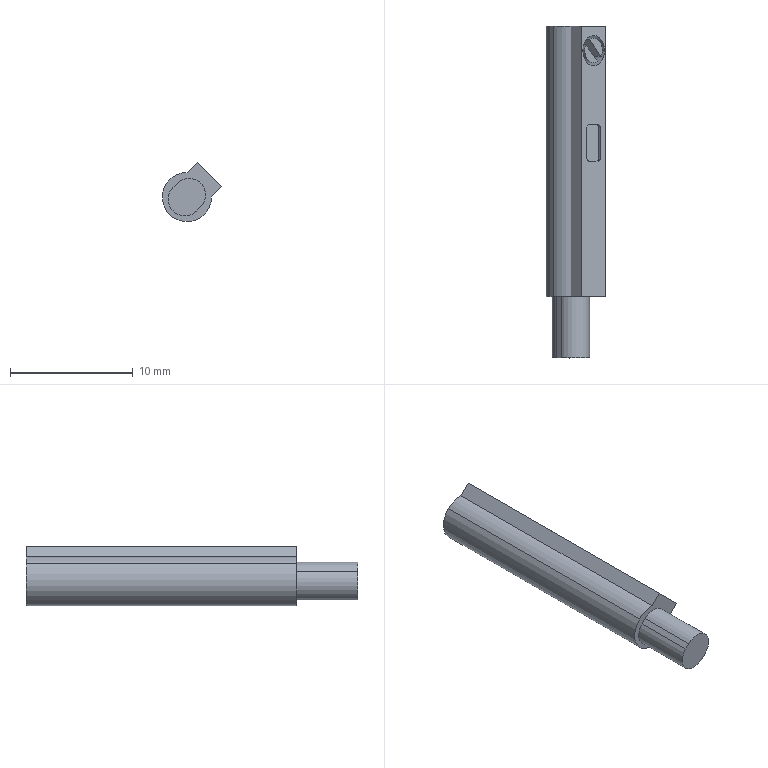Component | SolidWorks | BearingLiftingModule-1_CylinderLiftingModule-1_CDQ2B20-40DZ-L-M9B_0_0_0-1_D-M9B(CQ2_20)-1 | 1 solid | 32 faces | box 4.83 x 27 x 4.83 mm | volume 355 mm3 | plane 19 | cylinder 13 | commonest cylinder face diameters 0.6 x4 4 x3 2 x2 2.5 x2 2.7 x2
STEP:
#1=COLOUR_RGB('',0.7922,0.8196,0.9333);
#2=FILL_AREA_STYLE_COLOUR('',#1);
#3=FILL_AREA_STYLE('',(#2));
#4=SURFACE_STYLE_FILL_AREA(#3);
#5=SURFACE_SIDE_STYLE('',(#4));
#6=SURFACE_STYLE_USAGE(.BOTH.,#5);
#7=PRESENTATION_STYLE_ASSIGNMENT((#6));
#8=CARTESIAN_POINT('',(3.187,-4.024,1.713));
#9=VERTEX_POINT('',#8);
#10=CARTESIAN_POINT('',(3.147,-3.989,1.754));
#11=VERTEX_POINT('',#10);
#12=CARTESIAN_POINT('',(3.16,-4.024,1.741));
#13=DIRECTION('',(0.7071,0.,0.7071));
#14=DIRECTION('',(0.,-1.,0.));
#15=AXIS2_PLACEMENT_3D('',#12,#13,#14);
#16=CIRCLE('',#15,0.03937);
#17=EDGE_CURVE('',#9,#11,#16,.T.);
#18=ORIENTED_EDGE('',*,*,#17,.F.);
#19=CARTESIAN_POINT('',(3.146,-4.024,1.671));
#20=VERTEX_POINT('',#19);
#21=CARTESIAN_POINT('',(3.146,-4.024,1.671));
#22=DIRECTION('',(-0.7071,-0.,-0.7071));
#23=VECTOR('',#22,39.37);
#24=LINE('',#21,#23);
#25=EDGE_CURVE('',#9,#20,#24,.T.);
#26=ORIENTED_EDGE('',*,*,#25,.T.);
#27=CARTESIAN_POINT('',(3.09,-4.024,1.727));
#28=VERTEX_POINT('',#27);
#29=CARTESIAN_POINT('',(3.118,-4.024,1.699));
#30=DIRECTION('',(0.7071,0.,0.7071));
#31=DIRECTION('',(0.,-1.,0.));
#32=AXIS2_PLACEMENT_3D('',#29,#30,#31);
#33=CIRCLE('',#32,0.03937);
#34=EDGE_CURVE('',#20,#28,#33,.T.);
#35=ORIENTED_EDGE('',*,*,#34,.T.);
#36=CARTESIAN_POINT('',(3.132,-4.024,1.769));
#37=VERTEX_POINT('',#36);
#38=CARTESIAN_POINT('',(3.09,-4.024,1.727));
#39=DIRECTION('',(-0.7071,-0.,-0.7071));
#40=VECTOR('',#39,39.37);
#41=LINE('',#38,#40);
#42=EDGE_CURVE('',#37,#28,#41,.T.);
#43=ORIENTED_EDGE('',*,*,#42,.F.);
#44=CARTESIAN_POINT('',(3.135,-4.005,1.765));
#45=VERTEX_POINT('',#44);
#46=CARTESIAN_POINT('',(3.16,-4.024,1.741));
#47=DIRECTION('',(0.7071,0.,0.7071));
#48=DIRECTION('',(0.,-1.,0.));
#49=AXIS2_PLACEMENT_3D('',#46,#47,#48);
#50=CIRCLE('',#49,0.03937);
#51=EDGE_CURVE('',#45,#37,#50,.T.);
#52=ORIENTED_EDGE('',*,*,#51,.F.);
#53=CARTESIAN_POINT('',(3.107,-4.005,1.738));
#54=VERTEX_POINT('',#53);
#55=CARTESIAN_POINT('',(3.093,-4.005,1.724));
#56=DIRECTION('',(0.7071,0.,0.7071));
#57=VECTOR('',#56,39.37);
#58=LINE('',#55,#57);
#59=EDGE_CURVE('',#54,#45,#58,.T.);
#60=ORIENTED_EDGE('',*,*,#59,.F.);
#61=CARTESIAN_POINT('',(3.119,-3.989,1.726));
#62=VERTEX_POINT('',#61);
#63=CARTESIAN_POINT('',(3.132,-4.024,1.713));
#64=DIRECTION('',(-0.7071,-0.,-0.7071));
#65=DIRECTION('',(-0.7071,0.,0.7071));
#66=AXIS2_PLACEMENT_3D('',#63,#64,#65);
#67=CIRCLE('',#66,0.03937);
#68=EDGE_CURVE('',#54,#62,#67,.T.);
#69=ORIENTED_EDGE('',*,*,#68,.T.);
#70=CARTESIAN_POINT('',(3.105,-3.989,1.712));
#71=DIRECTION('',(-0.7071,-0.,-0.7071));
#72=VECTOR('',#71,39.37);
#73=LINE('',#70,#72);
#74=EDGE_CURVE('',#11,#62,#73,.T.);
#75=ORIENTED_EDGE('',*,*,#74,.F.);
#76=EDGE_LOOP('',(#18,#26,#35,#43,#52,#60,#69,#75));
#77=FACE_OUTER_BOUND('',#76,.T.);
#78=CARTESIAN_POINT('',(3.118,-4.024,1.699));
#79=DIRECTION('',(-0.7071,-0.,-0.7071));
#80=DIRECTION('',(-0.7071,0.,0.7071));
#81=AXIS2_PLACEMENT_3D('',#78,#79,#80);
#82=CYLINDRICAL_SURFACE('',#81,0.03937);
#83=ADVANCED_FACE('',(#77),#82,.T.);
#84=CARTESIAN_POINT('',(3.125,-4.024,1.775));
#85=VERTEX_POINT('',#84);
#86=CARTESIAN_POINT('',(3.194,-4.024,1.706));
#87=VERTEX_POINT('',#86);
#88=CARTESIAN_POINT('',(3.16,-4.024,1.741));
#89=DIRECTION('',(0.7071,0.,0.7071));
#90=DIRECTION('',(0.,-1.,0.));
#91=AXIS2_PLACEMENT_3D('',#88,#89,#90);
#92=CIRCLE('',#91,0.04921);
#93=EDGE_CURVE('',#85,#87,#92,.T.);
#94=ORIENTED_EDGE('',*,*,#93,.T.);
#95=CARTESIAN_POINT('',(3.153,-4.024,1.664));
#96=VERTEX_POINT('',#95);
#97=CARTESIAN_POINT('',(3.153,-4.024,1.664));
#98=DIRECTION('',(-0.7071,-0.,-0.7071));
#99=VECTOR('',#98,39.37);
#100=LINE('',#97,#99);
#101=EDGE_CURVE('',#87,#96,#100,.T.);
#102=ORIENTED_EDGE('',*,*,#101,.T.);
#103=CARTESIAN_POINT('',(3.083,-4.024,1.734));
#104=VERTEX_POINT('',#103);
#105=CARTESIAN_POINT('',(3.118,-4.024,1.699));
#106=DIRECTION('',(0.7071,0.,0.7071));
#107=DIRECTION('',(0.,-1.,0.));
#108=AXIS2_PLACEMENT_3D('',#105,#106,#107);
#109=CIRCLE('',#108,0.04921);
#110=EDGE_CURVE('',#104,#96,#109,.T.);
#111=ORIENTED_EDGE('',*,*,#110,.F.);
#112=CARTESIAN_POINT('',(3.083,-4.024,1.734));
#113=DIRECTION('',(-0.7071,-0.,-0.7071));
#114=VECTOR('',#113,39.37);
#115=LINE('',#112,#114);
#116=EDGE_CURVE('',#85,#104,#115,.T.);
#117=ORIENTED_EDGE('',*,*,#116,.F.);
#118=EDGE_LOOP('',(#94,#102,#111,#117));
#119=FACE_OUTER_BOUND('',#118,.T.);
#120=CARTESIAN_POINT('',(3.118,-4.024,1.699));
#121=DIRECTION('',(-0.7071,-0.,-0.7071));
#122=DIRECTION('',(-0.7071,0.,0.7071));
#123=AXIS2_PLACEMENT_3D('',#120,#121,#122);
#124=CYLINDRICAL_SURFACE('',#123,0.04921);
#125=ADVANCED_FACE('',(#119),#124,.F.);
#126=CARTESIAN_POINT('',(3.031,-3.945,1.724));
#127=VERTEX_POINT('',#126);
#128=CARTESIAN_POINT('',(3.143,-3.945,1.613));
#129=VERTEX_POINT('',#128);
#130=CARTESIAN_POINT('',(3.087,-3.945,1.668));
#131=DIRECTION('',(0.,-1.,0.));
#132=DIRECTION('',(0.7071,0.,-0.7071));
#133=AXIS2_PLACEMENT_3D('',#130,#131,#132);
#134=CIRCLE('',#133,0.07874);
#135=EDGE_CURVE('',#127,#129,#134,.T.);
#136=ORIENTED_EDGE('',*,*,#135,.T.);
#137=CARTESIAN_POINT('',(3.143,-4.811,1.613));
#138=VERTEX_POINT('',#137);
#139=CARTESIAN_POINT('',(3.143,-4.811,1.613));
#140=DIRECTION('',(0.,-1.,0.));
#141=VECTOR('',#140,39.37);
#142=LINE('',#139,#141);
#143=EDGE_CURVE('',#129,#138,#142,.T.);
#144=ORIENTED_EDGE('',*,*,#143,.T.);
#145=CARTESIAN_POINT('',(3.031,-4.811,1.724));
#146=VERTEX_POINT('',#145);
#147=CARTESIAN_POINT('',(3.087,-4.811,1.668));
#148=DIRECTION('',(0.,-1.,0.));
#149=DIRECTION('',(0.7071,0.,-0.7071));
#150=AXIS2_PLACEMENT_3D('',#147,#148,#149);
#151=CIRCLE('',#150,0.07874);
#152=EDGE_CURVE('',#146,#138,#151,.T.);
#153=ORIENTED_EDGE('',*,*,#152,.F.);
#154=CARTESIAN_POINT('',(3.031,-4.811,1.724));
#155=DIRECTION('',(0.,-1.,0.));
#156=VECTOR('',#155,39.37);
#157=LINE('',#154,#156);
#158=EDGE_CURVE('',#127,#146,#157,.T.);
#159=ORIENTED_EDGE('',*,*,#158,.F.);
#160=EDGE_LOOP('',(#136,#144,#153,#159));
#161=FACE_OUTER_BOUND('',#160,.T.);
#162=CARTESIAN_POINT('',(3.087,-4.811,1.668));
#163=DIRECTION('',(0.,-1.,0.));
#164=DIRECTION('',(-0.7071,0.,0.7071));
#165=AXIS2_PLACEMENT_3D('',#162,#163,#164);
#166=CYLINDRICAL_SURFACE('',#165,0.07874);
#167=ADVANCED_FACE('',(#161),#166,.T.);
#168=CARTESIAN_POINT('',(3.088,-3.945,1.747));
#169=VERTEX_POINT('',#168);
#170=CARTESIAN_POINT('',(3.087,-3.945,1.668));
#171=DIRECTION('',(0.,-1.,0.));
#172=DIRECTION('',(0.7071,0.,-0.7071));
#173=AXIS2_PLACEMENT_3D('',#170,#171,#172);
#174=CIRCLE('',#173,0.07874);
#175=EDGE_CURVE('',#169,#127,#174,.T.);
#176=ORIENTED_EDGE('',*,*,#175,.T.);
#177=ORIENTED_EDGE('',*,*,#158,.T.);
#178=CARTESIAN_POINT('',(3.088,-4.811,1.747));
#179=VERTEX_POINT('',#178);
#180=CARTESIAN_POINT('',(3.087,-4.811,1.668));
#181=DIRECTION('',(0.,-1.,0.));
#182=DIRECTION('',(0.7071,0.,-0.7071));
#183=AXIS2_PLACEMENT_3D('',#180,#181,#182);
#184=CIRCLE('',#183,0.07874);
#185=EDGE_CURVE('',#179,#146,#184,.T.);
#186=ORIENTED_EDGE('',*,*,#185,.F.);
#187=CARTESIAN_POINT('',(3.088,-4.811,1.747));
#188=DIRECTION('',(0.,1.,-0.));
#189=VECTOR('',#188,39.37);
#190=LINE('',#187,#189);
#191=EDGE_CURVE('',#179,#169,#190,.T.);
#192=ORIENTED_EDGE('',*,*,#191,.T.);
#193=EDGE_LOOP('',(#176,#177,#186,#192));
#194=FACE_OUTER_BOUND('',#193,.T.);
#195=CARTESIAN_POINT('',(3.087,-4.811,1.668));
#196=DIRECTION('',(0.,-1.,0.));
#197=DIRECTION('',(-0.7071,0.,0.7071));
#198=AXIS2_PLACEMENT_3D('',#195,#196,#197);
#199=CYLINDRICAL_SURFACE('',#198,0.07874);
#200=ADVANCED_FACE('',(#194),#199,.T.);
#201=CARTESIAN_POINT('',(3.184,-4.042,1.716));
#202=VERTEX_POINT('',#201);
#203=CARTESIAN_POINT('',(3.16,-4.024,1.741));
#204=DIRECTION('',(0.7071,0.,0.7071));
#205=DIRECTION('',(0.,-1.,0.));
#206=AXIS2_PLACEMENT_3D('',#203,#204,#205);
#207=CIRCLE('',#206,0.03937);
#208=EDGE_CURVE('',#202,#9,#207,.T.);
#209=ORIENTED_EDGE('',*,*,#208,.T.);
#210=ORIENTED_EDGE('',*,*,#17,.T.);
#211=CARTESIAN_POINT('',(3.186,-4.045,1.714));
#212=DIRECTION('',(-0.5,0.7071,0.5));
#213=VECTOR('',#212,39.37);
#214=LINE('',#211,#213);
#215=EDGE_CURVE('',#202,#11,#214,.T.);
#216=ORIENTED_EDGE('',*,*,#215,.F.);
#217=EDGE_LOOP('',(#209,#210,#216));
#218=FACE_OUTER_BOUND('',#217,.T.);
#219=CARTESIAN_POINT('',(3.199,-4.811,1.702));
#220=DIRECTION('',(-0.7071,-0.,-0.7071));
#221=DIRECTION('',(0.7071,-0.,-0.7071));
#222=AXIS2_PLACEMENT_3D('',#219,#220,#221);
#223=PLANE('',#222);
#224=ADVANCED_FACE('',(#218),#223,.F.);
#225=CARTESIAN_POINT('',(3.121,-3.945,1.78));
#226=VERTEX_POINT('',#225);
#227=CARTESIAN_POINT('',(3.121,-3.945,1.78));
#228=DIRECTION('',(-0.7071,-0.,-0.7071));
#229=VECTOR('',#228,39.37);
#230=LINE('',#227,#229);
#231=EDGE_CURVE('',#226,#169,#230,.T.);
#232=ORIENTED_EDGE('',*,*,#231,.T.);
#233=ORIENTED_EDGE('',*,*,#191,.F.);
#234=CARTESIAN_POINT('',(3.121,-4.811,1.78));
#235=VERTEX_POINT('',#234);
#236=CARTESIAN_POINT('',(3.121,-4.811,1.78));
#237=DIRECTION('',(-0.7071,-0.,-0.7071));
#238=VECTOR('',#237,39.37);
#239=LINE('',#236,#238);
#240=EDGE_CURVE('',#235,#179,#239,.T.);
#241=ORIENTED_EDGE('',*,*,#240,.F.);
#242=CARTESIAN_POINT('',(3.121,-4.811,1.78));
#243=DIRECTION('',(0.,1.,-0.));
#244=VECTOR('',#243,39.37);
#245=LINE('',#242,#244);
#246=EDGE_CURVE('',#235,#226,#245,.T.);
#247=ORIENTED_EDGE('',*,*,#246,.T.);
#248=EDGE_LOOP('',(#232,#233,#241,#247));
#249=FACE_OUTER_BOUND('',#248,.T.);
#250=CARTESIAN_POINT('',(3.121,-4.811,1.78));
#251=DIRECTION('',(0.7071,-0.,-0.7071));
#252=DIRECTION('',(-0.7071,-0.,-0.7071));
#253=AXIS2_PLACEMENT_3D('',#250,#251,#252);
#254=PLANE('',#253);
#255=ADVANCED_FACE('',(#249),#254,.F.);
#256=ORIENTED_EDGE('',*,*,#51,.T.);
#257=CARTESIAN_POINT('',(3.172,-4.058,1.728));
#258=VERTEX_POINT('',#257);
#259=CARTESIAN_POINT('',(3.16,-4.024,1.741));
#260=DIRECTION('',(0.7071,0.,0.7071));
#261=DIRECTION('',(0.,-1.,0.));
#262=AXIS2_PLACEMENT_3D('',#259,#260,#261);
#263=CIRCLE('',#262,0.03937);
#264=EDGE_CURVE('',#37,#258,#263,.T.);
#265=ORIENTED_EDGE('',*,*,#264,.T.);
#266=CARTESIAN_POINT('',(3.133,-4.002,1.767));
#267=DIRECTION('',(0.5,-0.7071,-0.5));
#268=VECTOR('',#267,39.37);
#269=LINE('',#266,#268);
#270=EDGE_CURVE('',#45,#258,#269,.T.);
#271=ORIENTED_EDGE('',*,*,#270,.F.);
#272=EDGE_LOOP('',(#256,#265,#271));
#273=FACE_OUTER_BOUND('',#272,.T.);
#274=CARTESIAN_POINT('',(3.199,-4.811,1.702));
#275=DIRECTION('',(-0.7071,-0.,-0.7071));
#276=DIRECTION('',(0.7071,-0.,-0.7071));
#277=AXIS2_PLACEMENT_3D('',#274,#275,#276);
#278=PLANE('',#277);
#279=ADVANCED_FACE('',(#273),#278,.F.);
#280=CARTESIAN_POINT('',(3.199,-3.945,1.702));
#281=VERTEX_POINT('',#280);
#282=CARTESIAN_POINT('',(3.199,-3.945,1.702));
#283=DIRECTION('',(-0.7071,0.,0.7071));
#284=VECTOR('',#283,39.37);
#285=LINE('',#282,#284);
#286=EDGE_CURVE('',#281,#226,#285,.T.);
#287=ORIENTED_EDGE('',*,*,#286,.T.);
#288=ORIENTED_EDGE('',*,*,#246,.F.);
#289=CARTESIAN_POINT('',(3.199,-4.811,1.702));
#290=VERTEX_POINT('',#289);
#291=CARTESIAN_POINT('',(3.199,-4.811,1.702));
#292=DIRECTION('',(-0.7071,0.,0.7071));
#293=VECTOR('',#292,39.37);
#294=LINE('',#291,#293);
#295=EDGE_CURVE('',#290,#235,#294,.T.);
#296=ORIENTED_EDGE('',*,*,#295,.F.);
#297=CARTESIAN_POINT('',(3.199,-4.811,1.702));
#298=DIRECTION('',(0.,1.,-0.));
#299=VECTOR('',#298,39.37);
#300=LINE('',#297,#299);
#301=EDGE_CURVE('',#290,#281,#300,.T.);
#302=ORIENTED_EDGE('',*,*,#301,.T.);
#303=EDGE_LOOP('',(#287,#288,#296,#302));
#304=FACE_OUTER_BOUND('',#303,.T.);
#305=CARTESIAN_POINT('',(3.173,-4.26,1.727));
#306=VERTEX_POINT('',#305);
#307=CARTESIAN_POINT('',(3.146,-4.26,1.755));
#308=VERTEX_POINT('',#307);
#309=CARTESIAN_POINT('',(3.173,-4.26,1.727));
#310=DIRECTION('',(-0.7071,0.,0.7071));
#311=VECTOR('',#310,39.37);
#312=LINE('',#309,#311);
#313=EDGE_CURVE('',#306,#308,#312,.T.);
#314=ORIENTED_EDGE('',*,*,#313,.F.);
#315=CARTESIAN_POINT('',(3.182,-4.272,1.718));
#316=VERTEX_POINT('',#315);
#317=CARTESIAN_POINT('',(3.173,-4.272,1.727));
#318=DIRECTION('',(0.7071,0.,0.7071));
#319=DIRECTION('',(0.,-1.,0.));
#320=AXIS2_PLACEMENT_3D('',#317,#318,#319);
#321=CIRCLE('',#320,0.01181);
#322=EDGE_CURVE('',#316,#306,#321,.T.);
#323=ORIENTED_EDGE('',*,*,#322,.F.);
#324=CARTESIAN_POINT('',(3.182,-4.366,1.718));
#325=VERTEX_POINT('',#324);
#326=CARTESIAN_POINT('',(3.182,-4.366,1.718));
#327=DIRECTION('',(0.,1.,-0.));
#328=VECTOR('',#327,39.37);
#329=LINE('',#326,#328);
#330=EDGE_CURVE('',#325,#316,#329,.T.);
#331=ORIENTED_EDGE('',*,*,#330,.F.);
#332=CARTESIAN_POINT('',(3.173,-4.378,1.727));
#333=VERTEX_POINT('',#332);
#334=CARTESIAN_POINT('',(3.173,-4.366,1.727));
#335=DIRECTION('',(0.7071,0.,0.7071));
#336=DIRECTION('',(0.,-1.,0.));
#337=AXIS2_PLACEMENT_3D('',#334,#335,#336);
#338=CIRCLE('',#337,0.01181);
#339=EDGE_CURVE('',#333,#325,#338,.T.);
#340=ORIENTED_EDGE('',*,*,#339,.F.);
#341=CARTESIAN_POINT('',(3.146,-4.378,1.755));
#342=VERTEX_POINT('',#341);
#343=CARTESIAN_POINT('',(3.146,-4.378,1.755));
#344=DIRECTION('',(0.7071,-0.,-0.7071));
#345=VECTOR('',#344,39.37);
#346=LINE('',#343,#345);
#347=EDGE_CURVE('',#342,#333,#346,.T.);
#348=ORIENTED_EDGE('',*,*,#347,.F.);
#349=CARTESIAN_POINT('',(3.137,-4.366,1.763));
#350=VERTEX_POINT('',#349);
#351=CARTESIAN_POINT('',(3.146,-4.366,1.755));
#352=DIRECTION('',(0.7071,0.,0.7071));
#353=DIRECTION('',(0.,-1.,0.));
#354=AXIS2_PLACEMENT_3D('',#351,#352,#353);
#355=CIRCLE('',#354,0.01181);
#356=EDGE_CURVE('',#350,#342,#355,.T.);
#357=ORIENTED_EDGE('',*,*,#356,.F.);
#358=CARTESIAN_POINT('',(3.137,-4.272,1.763));
#359=VERTEX_POINT('',#358);
#360=CARTESIAN_POINT('',(3.137,-4.272,1.763));
#361=DIRECTION('',(0.,-1.,0.));
#362=VECTOR('',#361,39.37);
#363=LINE('',#360,#362);
#364=EDGE_CURVE('',#359,#350,#363,.T.);
#365=ORIENTED_EDGE('',*,*,#364,.F.);
#366=CARTESIAN_POINT('',(3.146,-4.272,1.755));
#367=DIRECTION('',(0.7071,0.,0.7071));
#368=DIRECTION('',(0.,-1.,0.));
#369=AXIS2_PLACEMENT_3D('',#366,#367,#368);
#370=CIRCLE('',#369,0.01181);
#371=EDGE_CURVE('',#308,#359,#370,.T.);
#372=ORIENTED_EDGE('',*,*,#371,.F.);
#373=EDGE_LOOP('',(#314,#323,#331,#340,#348,#357,#365,#372));
#374=FACE_BOUND('',#373,.T.);
#375=ORIENTED_EDGE('',*,*,#93,.F.);
#376=CARTESIAN_POINT('',(3.16,-4.024,1.741));
#377=DIRECTION('',(0.7071,0.,0.7071));
#378=DIRECTION('',(0.,-1.,0.));
#379=AXIS2_PLACEMENT_3D('',#376,#377,#378);
#380=CIRCLE('',#379,0.04921);
#381=EDGE_CURVE('',#87,#85,#380,.T.);
#382=ORIENTED_EDGE('',*,*,#381,.F.);
#383=EDGE_LOOP('',(#375,#382));
#384=FACE_BOUND('',#383,.T.);
#385=CARTESIAN_POINT('',(3.199,-4.811,1.702));
#386=DIRECTION('',(-0.7071,-0.,-0.7071));
#387=DIRECTION('',(0.7071,-0.,-0.7071));
#388=AXIS2_PLACEMENT_3D('',#385,#386,#387);
#389=PLANE('',#388);
#390=ADVANCED_FACE('',(#304,#374,#384),#389,.F.);
#391=ORIENTED_EDGE('',*,*,#240,.T.);
#392=ORIENTED_EDGE('',*,*,#185,.T.);
#393=ORIENTED_EDGE('',*,*,#152,.T.);
#394=CARTESIAN_POINT('',(3.166,-4.811,1.669));
#395=VERTEX_POINT('',#394);
#396=CARTESIAN_POINT('',(3.087,-4.811,1.668));
#397=DIRECTION('',(0.,-1.,0.));
#398=DIRECTION('',(0.7071,0.,-0.7071));
#399=AXIS2_PLACEMENT_3D('',#396,#397,#398);
#400=CIRCLE('',#399,0.07874);
#401=EDGE_CURVE('',#138,#395,#400,.T.);
#402=ORIENTED_EDGE('',*,*,#401,.T.);
#403=CARTESIAN_POINT('',(3.166,-4.811,1.669));
#404=DIRECTION('',(0.7071,0.,0.7071));
#405=VECTOR('',#404,39.37);
#406=LINE('',#403,#405);
#407=EDGE_CURVE('',#395,#290,#406,.T.);
#408=ORIENTED_EDGE('',*,*,#407,.T.);
#409=ORIENTED_EDGE('',*,*,#295,.T.);
#410=EDGE_LOOP('',(#391,#392,#393,#402,#408,#409));
#411=FACE_OUTER_BOUND('',#410,.T.);
#412=CARTESIAN_POINT('',(3.118,-4.811,1.624));
#413=VERTEX_POINT('',#412);
#414=CARTESIAN_POINT('',(3.043,-4.811,1.699));
#415=VERTEX_POINT('',#414);
#416=CARTESIAN_POINT('',(3.08,-4.811,1.661));
#417=DIRECTION('',(0.,1.,-0.));
#418=DIRECTION('',(0.7071,0.,-0.7071));
#419=AXIS2_PLACEMENT_3D('',#416,#417,#418);
#420=CIRCLE('',#419,0.05315);
#421=EDGE_CURVE('',#413,#415,#420,.T.);
#422=ORIENTED_EDGE('',*,*,#421,.T.);
#423=CARTESIAN_POINT('',(3.057,-4.811,1.713));
#424=VERTEX_POINT('',#423);
#425=CARTESIAN_POINT('',(3.05,-4.811,1.706));
#426=DIRECTION('',(0.7071,0.,0.7071));
#427=VECTOR('',#426,39.37);
#428=LINE('',#425,#427);
#429=EDGE_CURVE('',#415,#424,#428,.T.);
#430=ORIENTED_EDGE('',*,*,#429,.T.);
#431=CARTESIAN_POINT('',(3.132,-4.811,1.638));
#432=VERTEX_POINT('',#431);
#433=CARTESIAN_POINT('',(3.094,-4.811,1.675));
#434=DIRECTION('',(0.,1.,-0.));
#435=DIRECTION('',(0.7071,0.,-0.7071));
#436=AXIS2_PLACEMENT_3D('',#433,#434,#435);
#437=CIRCLE('',#436,0.05315);
#438=EDGE_CURVE('',#424,#432,#437,.T.);
#439=ORIENTED_EDGE('',*,*,#438,.T.);
#440=CARTESIAN_POINT('',(3.125,-4.811,1.631));
#441=DIRECTION('',(-0.7071,-0.,-0.7071));
#442=VECTOR('',#441,39.37);
#443=LINE('',#440,#442);
#444=EDGE_CURVE('',#432,#413,#443,.T.);
#445=ORIENTED_EDGE('',*,*,#444,.T.);
#446=EDGE_LOOP('',(#422,#430,#439,#445));
#447=FACE_BOUND('',#446,.T.);
#448=CARTESIAN_POINT('',(3.087,-4.811,1.668));
#449=DIRECTION('',(0.,-1.,0.));
#450=DIRECTION('',(0.7071,0.,0.7071));
#451=AXIS2_PLACEMENT_3D('',#448,#449,#450);
#452=PLANE('',#451);
#453=ADVANCED_FACE('',(#411,#447),#452,.T.);
#454=CARTESIAN_POINT('',(3.166,-3.945,1.669));
#455=VERTEX_POINT('',#454);
#456=CARTESIAN_POINT('',(3.166,-3.945,1.669));
#457=DIRECTION('',(0.7071,0.,0.7071));
#458=VECTOR('',#457,39.37);
#459=LINE('',#456,#458);
#460=EDGE_CURVE('',#455,#281,#459,.T.);
#461=ORIENTED_EDGE('',*,*,#460,.T.);
#462=ORIENTED_EDGE('',*,*,#301,.F.);
#463=ORIENTED_EDGE('',*,*,#407,.F.);
#464=CARTESIAN_POINT('',(3.166,-4.811,1.669));
#465=DIRECTION('',(0.,1.,-0.));
#466=VECTOR('',#465,39.37);
#467=LINE('',#464,#466);
#468=EDGE_CURVE('',#395,#455,#467,.T.);
#469=ORIENTED_EDGE('',*,*,#468,.T.);
#470=EDGE_LOOP('',(#461,#462,#463,#469));
#471=FACE_OUTER_BOUND('',#470,.T.);
#472=CARTESIAN_POINT('',(3.166,-4.811,1.669));
#473=DIRECTION('',(-0.7071,0.,0.7071));
#474=DIRECTION('',(0.,-1.,0.));
#475=AXIS2_PLACEMENT_3D('',#472,#473,#474);
#476=PLANE('',#475);
#477=ADVANCED_FACE('',(#471),#476,.F.);
#478=ORIENTED_EDGE('',*,*,#143,.F.);
#479=CARTESIAN_POINT('',(3.087,-3.945,1.668));
#480=DIRECTION('',(0.,-1.,0.));
#481=DIRECTION('',(0.7071,0.,-0.7071));
#482=AXIS2_PLACEMENT_3D('',#479,#480,#481);
#483=CIRCLE('',#482,0.07874);
#484=EDGE_CURVE('',#129,#455,#483,.T.);
#485=ORIENTED_EDGE('',*,*,#484,.T.);
#486=ORIENTED_EDGE('',*,*,#468,.F.);
#487=ORIENTED_EDGE('',*,*,#401,.F.);
#488=EDGE_LOOP('',(#478,#485,#486,#487));
#489=FACE_OUTER_BOUND('',#488,.T.);
#490=CARTESIAN_POINT('',(3.087,-4.811,1.668));
#491=DIRECTION('',(0.,-1.,0.));
#492=DIRECTION('',(-0.7071,0.,0.7071));
#493=AXIS2_PLACEMENT_3D('',#490,#491,#492);
#494=CYLINDRICAL_SURFACE('',#493,0.07874);
#495=ADVANCED_FACE('',(#489),#494,.T.);
#496=ORIENTED_EDGE('',*,*,#231,.F.);
#497=ORIENTED_EDGE('',*,*,#286,.F.);
#498=ORIENTED_EDGE('',*,*,#460,.F.);
#499=ORIENTED_EDGE('',*,*,#484,.F.);
#500=ORIENTED_EDGE('',*,*,#135,.F.);
#501=ORIENTED_EDGE('',*,*,#175,.F.);
#502=EDGE_LOOP('',(#496,#497,#498,#499,#500,#501));
#503=FACE_OUTER_BOUND('',#502,.T.);
#504=CARTESIAN_POINT('',(3.087,-3.945,1.668));
#505=DIRECTION('',(0.,-1.,0.));
#506=DIRECTION('',(0.7071,0.,0.7071));
#507=AXIS2_PLACEMENT_3D('',#504,#505,#506);
#508=PLANE('',#507);
#509=ADVANCED_FACE('',(#503),#508,.F.);
#510=ORIENTED_EDGE('',*,*,#429,.F.);
#511=CARTESIAN_POINT('',(3.043,-5.008,1.699));
#512=VERTEX_POINT('',#511);
#513=CARTESIAN_POINT('',(3.043,-5.008,1.699));
#514=DIRECTION('',(0.,1.,-0.));
#515=VECTOR('',#514,39.37);
#516=LINE('',#513,#515);
#517=EDGE_CURVE('',#512,#415,#516,.T.);
#518=ORIENTED_EDGE('',*,*,#517,.F.);
#519=CARTESIAN_POINT('',(3.057,-5.008,1.713));
#520=VERTEX_POINT('',#519);
#521=CARTESIAN_POINT('',(3.057,-5.008,1.713));
#522=DIRECTION('',(-0.7071,-0.,-0.7071));
#523=VECTOR('',#522,39.37);
#524=LINE('',#521,#523);
#525=EDGE_CURVE('',#520,#512,#524,.T.);
#526=ORIENTED_EDGE('',*,*,#525,.F.);
#527=CARTESIAN_POINT('',(3.057,-5.008,1.713));
#528=DIRECTION('',(0.,1.,-0.));
#529=VECTOR('',#528,39.37);
#530=LINE('',#527,#529);
#531=EDGE_CURVE('',#520,#424,#530,.T.);
#532=ORIENTED_EDGE('',*,*,#531,.T.);
#533=EDGE_LOOP('',(#510,#518,#526,#532));
#534=FACE_OUTER_BOUND('',#533,.T.);
#535=CARTESIAN_POINT('',(3.057,-5.008,1.713));
#536=DIRECTION('',(0.7071,-0.,-0.7071));
#537=DIRECTION('',(-0.7071,-0.,-0.7071));
#538=AXIS2_PLACEMENT_3D('',#535,#536,#537);
#539=PLANE('',#538);
#540=ADVANCED_FACE('',(#534),#539,.F.);
#541=ORIENTED_EDGE('',*,*,#421,.F.);
#542=CARTESIAN_POINT('',(3.118,-5.008,1.624));
#543=VERTEX_POINT('',#542);
#544=CARTESIAN_POINT('',(3.118,-5.008,1.624));
#545=DIRECTION('',(0.,1.,-0.));
#546=VECTOR('',#545,39.37);
#547=LINE('',#544,#546);
#548=EDGE_CURVE('',#543,#413,#547,.T.);
#549=ORIENTED_EDGE('',*,*,#548,.F.);
#550=CARTESIAN_POINT('',(3.08,-5.008,1.661));
#551=DIRECTION('',(0.,-1.,0.));
#552=DIRECTION('',(0.7071,0.,-0.7071));
#553=AXIS2_PLACEMENT_3D('',#550,#551,#552);
#554=CIRCLE('',#553,0.05315);
#555=EDGE_CURVE('',#512,#543,#554,.T.);
#556=ORIENTED_EDGE('',*,*,#555,.F.);
#557=ORIENTED_EDGE('',*,*,#517,.T.);
#558=EDGE_LOOP('',(#541,#549,#556,#557));
#559=FACE_OUTER_BOUND('',#558,.T.);
#560=CARTESIAN_POINT('',(3.08,-5.008,1.661));
#561=DIRECTION('',(0.,-1.,0.));
#562=DIRECTION('',(-0.7071,0.,0.7071));
#563=AXIS2_PLACEMENT_3D('',#560,#561,#562);
#564=CYLINDRICAL_SURFACE('',#563,0.05315);
#565=ADVANCED_FACE('',(#559),#564,.T.);
#566=ORIENTED_EDGE('',*,*,#444,.F.);
#567=CARTESIAN_POINT('',(3.132,-5.008,1.638));
#568=VERTEX_POINT('',#567);
#569=CARTESIAN_POINT('',(3.132,-5.008,1.638));
#570=DIRECTION('',(0.,1.,-0.));
#571=VECTOR('',#570,39.37);
#572=LINE('',#569,#571);
#573=EDGE_CURVE('',#568,#432,#572,.T.);
#574=ORIENTED_EDGE('',*,*,#573,.F.);
#575=CARTESIAN_POINT('',(3.118,-5.008,1.624));
#576=DIRECTION('',(0.7071,0.,0.7071));
#577=VECTOR('',#576,39.37);
#578=LINE('',#575,#577);
#579=EDGE_CURVE('',#543,#568,#578,.T.);
#580=ORIENTED_EDGE('',*,*,#579,.F.);
#581=ORIENTED_EDGE('',*,*,#548,.T.);
#582=EDGE_LOOP('',(#566,#574,#580,#581));
#583=FACE_OUTER_BOUND('',#582,.T.);
#584=CARTESIAN_POINT('',(3.118,-5.008,1.624));
#585=DIRECTION('',(-0.7071,0.,0.7071));
#586=DIRECTION('',(0.,-1.,0.));
#587=AXIS2_PLACEMENT_3D('',#584,#585,#586);
#588=PLANE('',#587);
#589=ADVANCED_FACE('',(#583),#588,.F.);
#590=ORIENTED_EDGE('',*,*,#438,.F.);
#591=ORIENTED_EDGE('',*,*,#531,.F.);
#592=CARTESIAN_POINT('',(3.094,-5.008,1.675));
#593=DIRECTION('',(0.,-1.,0.));
#594=DIRECTION('',(0.7071,0.,-0.7071));
#595=AXIS2_PLACEMENT_3D('',#592,#593,#594);
#596=CIRCLE('',#595,0.05315);
#597=EDGE_CURVE('',#568,#520,#596,.T.);
#598=ORIENTED_EDGE('',*,*,#597,.F.);
#599=ORIENTED_EDGE('',*,*,#573,.T.);
#600=EDGE_LOOP('',(#590,#591,#598,#599));
#601=FACE_OUTER_BOUND('',#600,.T.);
#602=CARTESIAN_POINT('',(3.094,-5.008,1.675));
#603=DIRECTION('',(0.,-1.,0.));
#604=DIRECTION('',(-0.7071,0.,0.7071));
#605=AXIS2_PLACEMENT_3D('',#602,#603,#604);
#606=CYLINDRICAL_SURFACE('',#605,0.05315);
#607=ADVANCED_FACE('',(#601),#606,.T.);
#608=ORIENTED_EDGE('',*,*,#525,.T.);
#609=ORIENTED_EDGE('',*,*,#555,.T.);
#610=ORIENTED_EDGE('',*,*,#579,.T.);
#611=ORIENTED_EDGE('',*,*,#597,.T.);
#612=EDGE_LOOP('',(#608,#609,#610,#611));
#613=FACE_OUTER_BOUND('',#612,.T.);
#614=CARTESIAN_POINT('',(3.08,-5.008,1.661));
#615=DIRECTION('',(0.,-1.,0.));
#616=DIRECTION('',(0.7071,0.,0.7071));
#617=AXIS2_PLACEMENT_3D('',#614,#615,#616);
#618=PLANE('',#617);
#619=ADVANCED_FACE('',(#613),#618,.T.);
#620=ORIENTED_EDGE('',*,*,#101,.F.);
#621=ORIENTED_EDGE('',*,*,#381,.T.);
#622=ORIENTED_EDGE('',*,*,#116,.T.);
#623=CARTESIAN_POINT('',(3.118,-4.024,1.699));
#624=DIRECTION('',(0.7071,0.,0.7071));
#625=DIRECTION('',(0.,-1.,0.));
#626=AXIS2_PLACEMENT_3D('',#623,#624,#625);
#627=CIRCLE('',#626,0.04921);
#628=EDGE_CURVE('',#96,#104,#627,.T.);
#629=ORIENTED_EDGE('',*,*,#628,.F.);
#630=EDGE_LOOP('',(#620,#621,#622,#629));
#631=FACE_OUTER_BOUND('',#630,.T.);
#632=CARTESIAN_POINT('',(3.118,-4.024,1.699));
#633=DIRECTION('',(-0.7071,-0.,-0.7071));
#634=DIRECTION('',(-0.7071,0.,0.7071));
#635=AXIS2_PLACEMENT_3D('',#632,#633,#634);
#636=CYLINDRICAL_SURFACE('',#635,0.04921);
#637=ADVANCED_FACE('',(#631),#636,.F.);
#638=ORIENTED_EDGE('',*,*,#25,.F.);
#639=ORIENTED_EDGE('',*,*,#208,.F.);
#640=CARTESIAN_POINT('',(3.156,-4.042,1.688));
#641=VERTEX_POINT('',#640);
#642=CARTESIAN_POINT('',(3.142,-4.042,1.674));
#643=DIRECTION('',(0.7071,0.,0.7071));
#644=VECTOR('',#643,39.37);
#645=LINE('',#642,#644);
#646=EDGE_CURVE('',#641,#202,#645,.T.);
#647=ORIENTED_EDGE('',*,*,#646,.F.);
#648=CARTESIAN_POINT('',(3.145,-4.058,1.7));
#649=VERTEX_POINT('',#648);
#650=CARTESIAN_POINT('',(3.132,-4.024,1.713));
#651=DIRECTION('',(-0.7071,-0.,-0.7071));
#652=DIRECTION('',(-0.7071,0.,0.7071));
#653=AXIS2_PLACEMENT_3D('',#650,#651,#652);
#654=CIRCLE('',#653,0.03937);
#655=EDGE_CURVE('',#641,#649,#654,.T.);
#656=ORIENTED_EDGE('',*,*,#655,.T.);
#657=CARTESIAN_POINT('',(3.131,-4.058,1.686));
#658=DIRECTION('',(-0.7071,-0.,-0.7071));
#659=VECTOR('',#658,39.37);
#660=LINE('',#657,#659);
#661=EDGE_CURVE('',#258,#649,#660,.T.);
#662=ORIENTED_EDGE('',*,*,#661,.F.);
#663=ORIENTED_EDGE('',*,*,#264,.F.);
#664=ORIENTED_EDGE('',*,*,#42,.T.);
#665=CARTESIAN_POINT('',(3.118,-4.024,1.699));
#666=DIRECTION('',(0.7071,0.,0.7071));
#667=DIRECTION('',(0.,-1.,0.));
#668=AXIS2_PLACEMENT_3D('',#665,#666,#667);
#669=CIRCLE('',#668,0.03937);
#670=EDGE_CURVE('',#28,#20,#669,.T.);
#671=ORIENTED_EDGE('',*,*,#670,.T.);
#672=EDGE_LOOP('',(#638,#639,#647,#656,#662,#663,#664,#671));
#673=FACE_OUTER_BOUND('',#672,.T.);
#674=CARTESIAN_POINT('',(3.118,-4.024,1.699));
#675=DIRECTION('',(-0.7071,-0.,-0.7071));
#676=DIRECTION('',(-0.7071,0.,0.7071));
#677=AXIS2_PLACEMENT_3D('',#674,#675,#676);
#678=CYLINDRICAL_SURFACE('',#677,0.03937);
#679=ADVANCED_FACE('',(#673),#678,.T.);
#680=ORIENTED_EDGE('',*,*,#110,.T.);
#681=ORIENTED_EDGE('',*,*,#628,.T.);
#682=EDGE_LOOP('',(#680,#681));
#683=FACE_OUTER_BOUND('',#682,.T.);
#684=ORIENTED_EDGE('',*,*,#670,.F.);
#685=ORIENTED_EDGE('',*,*,#34,.F.);
#686=EDGE_LOOP('',(#684,#685));
#687=FACE_BOUND('',#686,.T.);
#688=CARTESIAN_POINT('',(3.118,-4.024,1.699));
#689=DIRECTION('',(0.7071,0.,0.7071));
#690=DIRECTION('',(0.,-1.,0.));
#691=AXIS2_PLACEMENT_3D('',#688,#689,#690);
#692=PLANE('',#691);
#693=ADVANCED_FACE('',(#683,#687),#692,.T.);
#694=ORIENTED_EDGE('',*,*,#74,.T.);
#695=CARTESIAN_POINT('',(3.158,-4.045,1.686));
#696=DIRECTION('',(-0.5,0.7071,0.5));
#697=VECTOR('',#696,39.37);
#698=LINE('',#695,#697);
#699=EDGE_CURVE('',#641,#62,#698,.T.);
#700=ORIENTED_EDGE('',*,*,#699,.F.);
#701=ORIENTED_EDGE('',*,*,#646,.T.);
#702=ORIENTED_EDGE('',*,*,#215,.T.);
#703=EDGE_LOOP('',(#694,#700,#701,#702));
#704=FACE_OUTER_BOUND('',#703,.T.);
#705=CARTESIAN_POINT('',(3.158,-4.045,1.686));
#706=DIRECTION('',(0.5,0.7071,-0.5));
#707=DIRECTION('',(-0.5,0.7071,0.5));
#708=AXIS2_PLACEMENT_3D('',#705,#706,#707);
#709=PLANE('',#708);
#710=ADVANCED_FACE('',(#704),#709,.F.);
#711=ORIENTED_EDGE('',*,*,#661,.T.);
#712=CARTESIAN_POINT('',(3.105,-4.002,1.74));
#713=DIRECTION('',(0.5,-0.7071,-0.5));
#714=VECTOR('',#713,39.37);
#715=LINE('',#712,#714);
#716=EDGE_CURVE('',#54,#649,#715,.T.);
#717=ORIENTED_EDGE('',*,*,#716,.F.);
#718=ORIENTED_EDGE('',*,*,#59,.T.);
#719=ORIENTED_EDGE('',*,*,#270,.T.);
#720=EDGE_LOOP('',(#711,#717,#718,#719));
#721=FACE_OUTER_BOUND('',#720,.T.);
#722=CARTESIAN_POINT('',(3.105,-4.002,1.74));
#723=DIRECTION('',(-0.5,-0.7071,0.5));
#724=DIRECTION('',(-0.7071,-0.,-0.7071));
#725=AXIS2_PLACEMENT_3D('',#722,#723,#724);
#726=PLANE('',#725);
#727=ADVANCED_FACE('',(#721),#726,.F.);
#728=ORIENTED_EDGE('',*,*,#716,.T.);
#729=ORIENTED_EDGE('',*,*,#655,.F.);
#730=ORIENTED_EDGE('',*,*,#699,.T.);
#731=ORIENTED_EDGE('',*,*,#68,.F.);
#732=EDGE_LOOP('',(#728,#729,#730,#731));
#733=FACE_OUTER_BOUND('',#732,.T.);
#734=CARTESIAN_POINT('',(3.132,-4.024,1.713));
#735=DIRECTION('',(0.7071,0.,0.7071));
#736=DIRECTION('',(0.,-1.,0.));
#737=AXIS2_PLACEMENT_3D('',#734,#735,#736);
#738=PLANE('',#737);
#739=ADVANCED_FACE('',(#733),#738,.T.);
#740=ORIENTED_EDGE('',*,*,#322,.T.);
#741=CARTESIAN_POINT('',(3.168,-4.26,1.721));
#742=VERTEX_POINT('',#741);
#743=CARTESIAN_POINT('',(3.168,-4.26,1.721));
#744=DIRECTION('',(0.7071,0.,0.7071));
#745=VECTOR('',#744,39.37);
#746=LINE('',#743,#745);
#747=EDGE_CURVE('',#742,#306,#746,.T.);
#748=ORIENTED_EDGE('',*,*,#747,.F.);
#749=CARTESIAN_POINT('',(3.176,-4.272,1.713));
#750=VERTEX_POINT('',#749);
#751=CARTESIAN_POINT('',(3.168,-4.272,1.721));
#752=DIRECTION('',(0.7071,0.,0.7071));
#753=DIRECTION('',(0.,-1.,0.));
#754=AXIS2_PLACEMENT_3D('',#751,#752,#753);
#755=CIRCLE('',#754,0.01181);
#756=EDGE_CURVE('',#750,#742,#755,.T.);
#757=ORIENTED_EDGE('',*,*,#756,.F.);
#758=CARTESIAN_POINT('',(3.176,-4.272,1.713));
#759=DIRECTION('',(0.7071,0.,0.7071));
#760=VECTOR('',#759,39.37);
#761=LINE('',#758,#760);
#762=EDGE_CURVE('',#750,#316,#761,.T.);
#763=ORIENTED_EDGE('',*,*,#762,.T.);
#764=EDGE_LOOP('',(#740,#748,#757,#763));
#765=FACE_OUTER_BOUND('',#764,.T.);
#766=CARTESIAN_POINT('',(3.168,-4.272,1.721));
#767=DIRECTION('',(-0.7071,-0.,-0.7071));
#768=DIRECTION('',(-0.7071,0.,0.7071));
#769=AXIS2_PLACEMENT_3D('',#766,#767,#768);
#770=CYLINDRICAL_SURFACE('',#769,0.01181);
#771=ADVANCED_FACE('',(#765),#770,.F.);
#772=ORIENTED_EDGE('',*,*,#313,.T.);
#773=CARTESIAN_POINT('',(3.14,-4.26,1.749));
#774=VERTEX_POINT('',#773);
#775=CARTESIAN_POINT('',(3.14,-4.26,1.749));
#776=DIRECTION('',(0.7071,0.,0.7071));
#777=VECTOR('',#776,39.37);
#778=LINE('',#775,#777);
#779=EDGE_CURVE('',#774,#308,#778,.T.);
#780=ORIENTED_EDGE('',*,*,#779,.F.);
#781=CARTESIAN_POINT('',(3.168,-4.26,1.721));
#782=DIRECTION('',(-0.7071,0.,0.7071));
#783=VECTOR('',#782,39.37);
#784=LINE('',#781,#783);
#785=EDGE_CURVE('',#742,#774,#784,.T.);
#786=ORIENTED_EDGE('',*,*,#785,.F.);
#787=ORIENTED_EDGE('',*,*,#747,.T.);
#788=EDGE_LOOP('',(#772,#780,#786,#787));
#789=FACE_OUTER_BOUND('',#788,.T.);
#790=CARTESIAN_POINT('',(3.168,-4.26,1.721));
#791=DIRECTION('',(0.,1.,-0.));
#792=DIRECTION('',(-0.7071,0.,0.7071));
#793=AXIS2_PLACEMENT_3D('',#790,#791,#792);
#794=PLANE('',#793);
#795=ADVANCED_FACE('',(#789),#794,.F.);
#796=ORIENTED_EDGE('',*,*,#371,.T.);
#797=CARTESIAN_POINT('',(3.132,-4.272,1.757));
#798=VERTEX_POINT('',#797);
#799=CARTESIAN_POINT('',(3.132,-4.272,1.757));
#800=DIRECTION('',(0.7071,0.,0.7071));
#801=VECTOR('',#800,39.37);
#802=LINE('',#799,#801);
#803=EDGE_CURVE('',#798,#359,#802,.T.);
#804=ORIENTED_EDGE('',*,*,#803,.F.);
#805=CARTESIAN_POINT('',(3.14,-4.272,1.749));
#806=DIRECTION('',(0.7071,0.,0.7071));
#807=DIRECTION('',(0.,-1.,0.));
#808=AXIS2_PLACEMENT_3D('',#805,#806,#807);
#809=CIRCLE('',#808,0.01181);
#810=EDGE_CURVE('',#774,#798,#809,.T.);
#811=ORIENTED_EDGE('',*,*,#810,.F.);
#812=ORIENTED_EDGE('',*,*,#779,.T.);
#813=EDGE_LOOP('',(#796,#804,#811,#812));
#814=FACE_OUTER_BOUND('',#813,.T.);
#815=CARTESIAN_POINT('',(3.14,-4.272,1.749));
#816=DIRECTION('',(-0.7071,-0.,-0.7071));
#817=DIRECTION('',(-0.7071,0.,0.7071));
#818=AXIS2_PLACEMENT_3D('',#815,#816,#817);
#819=CYLINDRICAL_SURFACE('',#818,0.01181);
#820=ADVANCED_FACE('',(#814),#819,.F.);
#821=ORIENTED_EDGE('',*,*,#364,.T.);
#822=CARTESIAN_POINT('',(3.132,-4.366,1.757));
#823=VERTEX_POINT('',#822);
#824=CARTESIAN_POINT('',(3.132,-4.366,1.757));
#825=DIRECTION('',(0.7071,0.,0.7071));
#826=VECTOR('',#825,39.37);
#827=LINE('',#824,#826);
#828=EDGE_CURVE('',#823,#350,#827,.T.);
#829=ORIENTED_EDGE('',*,*,#828,.F.);
#830=CARTESIAN_POINT('',(3.132,-4.272,1.757));
#831=DIRECTION('',(0.,-1.,0.));
#832=VECTOR('',#831,39.37);
#833=LINE('',#830,#832);
#834=EDGE_CURVE('',#798,#823,#833,.T.);
#835=ORIENTED_EDGE('',*,*,#834,.F.);
#836=ORIENTED_EDGE('',*,*,#803,.T.);
#837=EDGE_LOOP('',(#821,#829,#835,#836));
#838=FACE_OUTER_BOUND('',#837,.T.);
#839=CARTESIAN_POINT('',(3.132,-4.272,1.757));
#840=DIRECTION('',(-0.7071,0.,0.7071));
#841=DIRECTION('',(0.,-1.,0.));
#842=AXIS2_PLACEMENT_3D('',#839,#840,#841);
#843=PLANE('',#842);
#844=ADVANCED_FACE('',(#838),#843,.F.);
#845=ORIENTED_EDGE('',*,*,#356,.T.);
#846=CARTESIAN_POINT('',(3.14,-4.378,1.749));
#847=VERTEX_POINT('',#846);
#848=CARTESIAN_POINT('',(3.14,-4.378,1.749));
#849=DIRECTION('',(0.7071,0.,0.7071));
#850=VECTOR('',#849,39.37);
#851=LINE('',#848,#850);
#852=EDGE_CURVE('',#847,#342,#851,.T.);
#853=ORIENTED_EDGE('',*,*,#852,.F.);
#854=CARTESIAN_POINT('',(3.14,-4.366,1.749));
#855=DIRECTION('',(0.7071,0.,0.7071));
#856=DIRECTION('',(0.,-1.,0.));
#857=AXIS2_PLACEMENT_3D('',#854,#855,#856);
#858=CIRCLE('',#857,0.01181);
#859=EDGE_CURVE('',#823,#847,#858,.T.);
#860=ORIENTED_EDGE('',*,*,#859,.F.);
#861=ORIENTED_EDGE('',*,*,#828,.T.);
#862=EDGE_LOOP('',(#845,#853,#860,#861));
#863=FACE_OUTER_BOUND('',#862,.T.);
#864=CARTESIAN_POINT('',(3.14,-4.366,1.749));
#865=DIRECTION('',(-0.7071,-0.,-0.7071));
#866=DIRECTION('',(-0.7071,0.,0.7071));
#867=AXIS2_PLACEMENT_3D('',#864,#865,#866);
#868=CYLINDRICAL_SURFACE('',#867,0.01181);
#869=ADVANCED_FACE('',(#863),#868,.F.);
#870=ORIENTED_EDGE('',*,*,#347,.T.);
#871=CARTESIAN_POINT('',(3.168,-4.378,1.721));
#872=VERTEX_POINT('',#871);
#873=CARTESIAN_POINT('',(3.168,-4.378,1.721));
#874=DIRECTION('',(0.7071,0.,0.7071));
#875=VECTOR('',#874,39.37);
#876=LINE('',#873,#875);
#877=EDGE_CURVE('',#872,#333,#876,.T.);
#878=ORIENTED_EDGE('',*,*,#877,.F.);
#879=CARTESIAN_POINT('',(3.14,-4.378,1.749));
#880=DIRECTION('',(0.7071,-0.,-0.7071));
#881=VECTOR('',#880,39.37);
#882=LINE('',#879,#881);
#883=EDGE_CURVE('',#847,#872,#882,.T.);
#884=ORIENTED_EDGE('',*,*,#883,.F.);
#885=ORIENTED_EDGE('',*,*,#852,.T.);
#886=EDGE_LOOP('',(#870,#878,#884,#885));
#887=FACE_OUTER_BOUND('',#886,.T.);
#888=CARTESIAN_POINT('',(3.14,-4.378,1.749));
#889=DIRECTION('',(0.,-1.,0.));
#890=DIRECTION('',(0.7071,0.,0.7071));
#891=AXIS2_PLACEMENT_3D('',#888,#889,#890);
#892=PLANE('',#891);
#893=ADVANCED_FACE('',(#887),#892,.F.);
#894=ORIENTED_EDGE('',*,*,#339,.T.);
#895=CARTESIAN_POINT('',(3.176,-4.366,1.713));
#896=VERTEX_POINT('',#895);
#897=CARTESIAN_POINT('',(3.176,-4.366,1.713));
#898=DIRECTION('',(0.7071,0.,0.7071));
#899=VECTOR('',#898,39.37);
#900=LINE('',#897,#899);
#901=EDGE_CURVE('',#896,#325,#900,.T.);
#902=ORIENTED_EDGE('',*,*,#901,.F.);
#903=CARTESIAN_POINT('',(3.168,-4.366,1.721));
#904=DIRECTION('',(0.7071,0.,0.7071));
#905=DIRECTION('',(0.,-1.,0.));
#906=AXIS2_PLACEMENT_3D('',#903,#904,#905);
#907=CIRCLE('',#906,0.01181);
#908=EDGE_CURVE('',#872,#896,#907,.T.);
#909=ORIENTED_EDGE('',*,*,#908,.F.);
#910=ORIENTED_EDGE('',*,*,#877,.T.);
#911=EDGE_LOOP('',(#894,#902,#909,#910));
#912=FACE_OUTER_BOUND('',#911,.T.);
#913=CARTESIAN_POINT('',(3.168,-4.366,1.721));
#914=DIRECTION('',(-0.7071,-0.,-0.7071));
#915=DIRECTION('',(-0.7071,0.,0.7071));
#916=AXIS2_PLACEMENT_3D('',#913,#914,#915);
#917=CYLINDRICAL_SURFACE('',#916,0.01181);
#918=ADVANCED_FACE('',(#912),#917,.F.);
#919=ORIENTED_EDGE('',*,*,#330,.T.);
#920=ORIENTED_EDGE('',*,*,#762,.F.);
#921=CARTESIAN_POINT('',(3.176,-4.366,1.713));
#922=DIRECTION('',(0.,1.,-0.));
#923=VECTOR('',#922,39.37);
#924=LINE('',#921,#923);
#925=EDGE_CURVE('',#896,#750,#924,.T.);
#926=ORIENTED_EDGE('',*,*,#925,.F.);
#927=ORIENTED_EDGE('',*,*,#901,.T.);
#928=EDGE_LOOP('',(#919,#920,#926,#927));
#929=FACE_OUTER_BOUND('',#928,.T.);
#930=CARTESIAN_POINT('',(3.176,-4.366,1.713));
#931=DIRECTION('',(0.7071,-0.,-0.7071));
#932=DIRECTION('',(-0.7071,-0.,-0.7071));
#933=AXIS2_PLACEMENT_3D('',#930,#931,#932);
#934=PLANE('',#933);
#935=ADVANCED_FACE('',(#929),#934,.F.);
#936=ORIENTED_EDGE('',*,*,#756,.T.);
#937=ORIENTED_EDGE('',*,*,#785,.T.);
#938=ORIENTED_EDGE('',*,*,#810,.T.);
#939=ORIENTED_EDGE('',*,*,#834,.T.);
#940=ORIENTED_EDGE('',*,*,#859,.T.);
#941=ORIENTED_EDGE('',*,*,#883,.T.);
#942=ORIENTED_EDGE('',*,*,#908,.T.);
#943=ORIENTED_EDGE('',*,*,#925,.T.);
#944=EDGE_LOOP('',(#936,#937,#938,#939,#940,#941,#942,#943));
#945=FACE_OUTER_BOUND('',#944,.T.);
#946=CARTESIAN_POINT('',(3.168,-4.272,1.721));
#947=DIRECTION('',(0.7071,0.,0.7071));
#948=DIRECTION('',(0.,-1.,0.));
#949=AXIS2_PLACEMENT_3D('',#946,#947,#948);
#950=PLANE('',#949);
#951=ADVANCED_FACE('',(#945),#950,.T.);
#952=CLOSED_SHELL('',(#83,#125,#167,#200,#224,#255,#279,#390,#453,#477,#495,#509,#540,#565,#589,#607,#619,#637,#679,#693,#710,#727,#739,#771,#795,#820,#844,#869,#893,#918,#935,#951));
#953=MANIFOLD_SOLID_BREP('',#952);
#954=STYLED_ITEM('',(#7),#953);
#955=PRESENTATION_LAYER_ASSIGNMENT('','',(#954));
#956=(LENGTH_UNIT()NAMED_UNIT(*)SI_UNIT($,.METRE.));
#957=LENGTH_MEASURE_WITH_UNIT(LENGTH_MEASURE(0.0254),#956);
#958=DIMENSIONAL_EXPONENTS(1.,0.,0.,0.,0.,0.,0.);
#959=(CONVERSION_BASED_UNIT('',#957)LENGTH_UNIT()NAMED_UNIT(#958));
#960=UNCERTAINTY_MEASURE_WITH_UNIT(LENGTH_MEASURE(0.00001),#959,'','');
#961=(NAMED_UNIT(*)PLANE_ANGLE_UNIT()SI_UNIT($,.RADIAN.));
#962=(NAMED_UNIT(*)SI_UNIT($,.STERADIAN.)SOLID_ANGLE_UNIT());
#963=(GEOMETRIC_REPRESENTATION_CONTEXT(3)GLOBAL_UNCERTAINTY_ASSIGNED_CONTEXT((#960))GLOBAL_UNIT_ASSIGNED_CONTEXT((#959,#961,#962))REPRESENTATION_CONTEXT('',''));
#964=MECHANICAL_DESIGN_GEOMETRIC_PRESENTATION_REPRESENTATION('',(#954),#963);
#965=CARTESIAN_POINT('',(0.,0.,0.));
#966=DIRECTION('',(0.,0.,1.));
#967=DIRECTION('',(1.,0.,0.));
#968=AXIS2_PLACEMENT_3D('',#965,#966,#967);
#969=(LENGTH_UNIT()NAMED_UNIT(*)SI_UNIT($,.METRE.));
#970=LENGTH_MEASURE_WITH_UNIT(LENGTH_MEASURE(0.0254),#969);
#971=DIMENSIONAL_EXPONENTS(1.,0.,0.,0.,0.,0.,0.);
#972=(CONVERSION_BASED_UNIT('',#970)LENGTH_UNIT()NAMED_UNIT(#971));
#973=UNCERTAINTY_MEASURE_WITH_UNIT(LENGTH_MEASURE(0.00001),#972,'','');
#974=(NAMED_UNIT(*)PLANE_ANGLE_UNIT()SI_UNIT($,.RADIAN.));
#975=(NAMED_UNIT(*)SI_UNIT($,.STERADIAN.)SOLID_ANGLE_UNIT());
#976=(GEOMETRIC_REPRESENTATION_CONTEXT(3)GLOBAL_UNCERTAINTY_ASSIGNED_CONTEXT((#973))GLOBAL_UNIT_ASSIGNED_CONTEXT((#972,#974,#975))REPRESENTATION_CONTEXT('',''));
#977=ADVANCED_BREP_SHAPE_REPRESENTATION('',(#953,#968),#976);